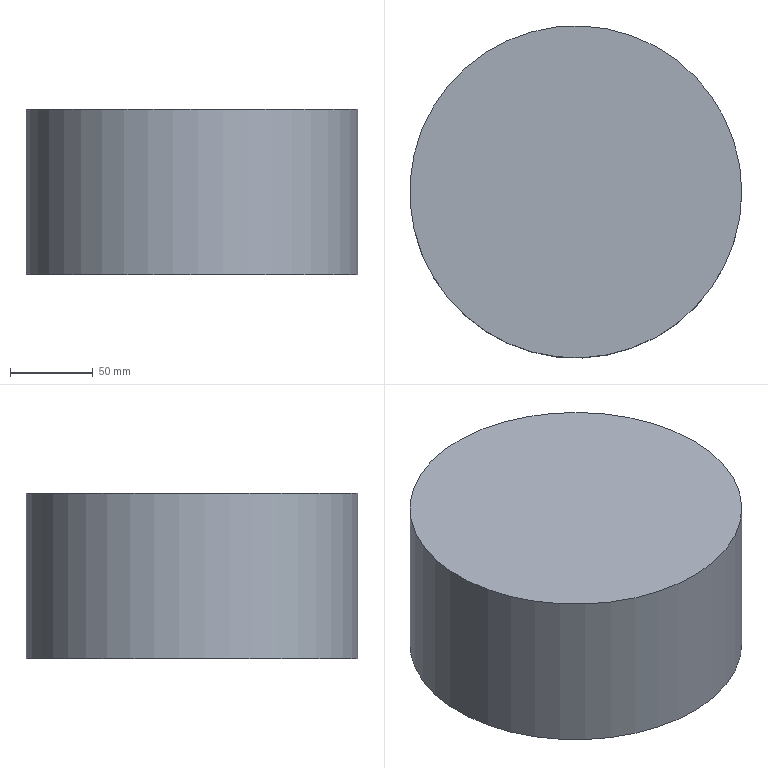CAM job | NX | mm | 3-axis | 1 set-up | 1 operations | part box 200 x 200 x 100
set-up 1
1. Z-Level Milling | Mill Mill5 D10 | ZLEVEL_PROFILE | path 11603.798 mm | 4.607 min